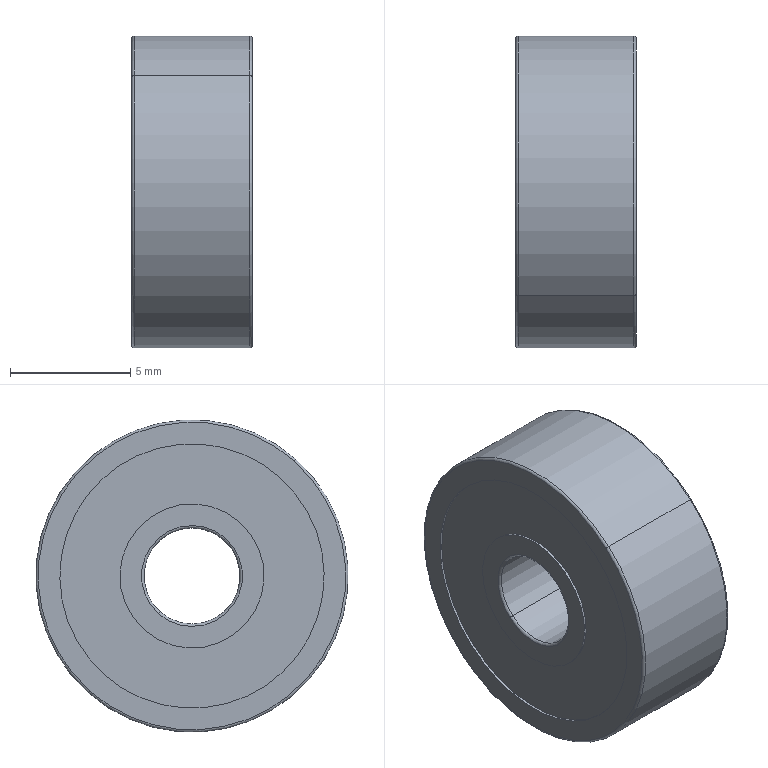Component | SolidWorks | DeepGrooveBallBearing624-2Z-1 | 1 solid | 26 faces | box 5 x 13 x 13 mm | volume 587 mm3 | cylinder 12 | torus 8 | plane 6 | commonest cylinder face diameters 11 x4 6 x4 13 x2 4 x2
build123d program:
from build123d import *

# Parameters (mm, degrees)
FILLET1_R = 0.1


with BuildPart() as part:
    # Sketch1 → Revolve1 (revolve)
    with BuildSketch(Plane.XY, mode=Mode.PRIVATE) as revolve1_sk:
        Polygon((-2.5, 6.5), (2.5, 6.5), (2.5, 5.5), (2.4, 5.5), (2.4, 3), (2.5, 3), (2.5, 2), (-2.5, 2), (-2.5, 3), (-2.4, 3), (-2.4, 5.5), (-2.5, 5.5), align=None)
    revolve(revolve1_sk.sketch.rotate(Axis((0, 0, 0), (1, 0, 0)), 90), axis=Axis((0, 0, 0), (1, 0, 0)))

    # Fillet1
    fillet1_edges = [part.edges().sort_by_distance(p)[0] for p in [
        (-2.5, 0, -2),
        (2.5, 0, -2),
        (2.5, 0, -6.5),
        (-2.5, 0, -6.5),
    ]]
    fillet(fillet1_edges, radius=FILLET1_R)


solid = part.part

# Placed as in the assembly
solid = solid.moved(Location((-0.3, -4.5, -27.446), (0, 0, 0)))
STEP:
#1=COLOUR_RGB('',0.7922,0.8196,0.9333);
#2=FILL_AREA_STYLE_COLOUR('',#1);
#3=FILL_AREA_STYLE('',(#2));
#4=SURFACE_STYLE_FILL_AREA(#3);
#5=SURFACE_SIDE_STYLE('',(#4));
#6=SURFACE_STYLE_USAGE(.BOTH.,#5);
#7=PRESENTATION_STYLE_ASSIGNMENT((#6));
#8=CARTESIAN_POINT('',(0.08661,-0.009757,-1.269));
#9=VERTEX_POINT('',#8);
#10=CARTESIAN_POINT('',(0.08661,-0.3446,-0.8922));
#11=VERTEX_POINT('',#10);
#12=CARTESIAN_POINT('',(0.08661,-0.1772,-1.081));
#13=DIRECTION('',(1.,-0.,-0.));
#14=DIRECTION('',(0.,-0.6644,0.7474));
#15=AXIS2_PLACEMENT_3D('',#12,#13,#14);
#16=CIRCLE('',#15,0.252);
#17=EDGE_CURVE('',#9,#11,#16,.T.);
#18=ORIENTED_EDGE('',*,*,#17,.F.);
#19=CARTESIAN_POINT('',(0.08268,-0.007141,-1.272));
#20=VERTEX_POINT('',#19);
#21=CARTESIAN_POINT('',(0.08268,-0.009757,-1.269));
#22=DIRECTION('',(0.,0.7474,0.6644));
#23=DIRECTION('',(0.,-0.6644,0.7474));
#24=AXIS2_PLACEMENT_3D('',#21,#22,#23);
#25=CIRCLE('',#24,0.003937);
#26=EDGE_CURVE('',#9,#20,#25,.T.);
#27=ORIENTED_EDGE('',*,*,#26,.T.);
#28=CARTESIAN_POINT('',(0.08268,-0.3472,-0.8893));
#29=VERTEX_POINT('',#28);
#30=CARTESIAN_POINT('',(0.08268,-0.1772,-1.081));
#31=DIRECTION('',(-1.,0.,0.));
#32=DIRECTION('',(0.,-0.6644,0.7474));
#33=AXIS2_PLACEMENT_3D('',#30,#31,#32);
#34=CIRCLE('',#33,0.2559);
#35=EDGE_CURVE('',#29,#20,#34,.T.);
#36=ORIENTED_EDGE('',*,*,#35,.F.);
#37=CARTESIAN_POINT('',(0.08268,-0.3446,-0.8922));
#38=DIRECTION('',(-0.,-0.7474,-0.6644));
#39=DIRECTION('',(0.,0.6644,-0.7474));
#40=AXIS2_PLACEMENT_3D('',#37,#38,#39);
#41=CIRCLE('',#40,0.003937);
#42=EDGE_CURVE('',#11,#29,#41,.T.);
#43=ORIENTED_EDGE('',*,*,#42,.F.);
#44=EDGE_LOOP('',(#18,#27,#36,#43));
#45=FACE_OUTER_BOUND('',#44,.T.);
#46=CARTESIAN_POINT('',(0.08268,-0.1772,-1.081));
#47=DIRECTION('',(-1.,0.,0.));
#48=DIRECTION('',(0.,-0.6644,0.7474));
#49=AXIS2_PLACEMENT_3D('',#46,#47,#48);
#50=TOROIDAL_SURFACE('',#49,0.252,0.003937);
#51=ADVANCED_FACE('',(#45),#50,.T.);
#52=CARTESIAN_POINT('',(-0.1102,-0.3446,-0.8922));
#53=VERTEX_POINT('',#52);
#54=CARTESIAN_POINT('',(-0.1102,-0.009757,-1.269));
#55=VERTEX_POINT('',#54);
#56=CARTESIAN_POINT('',(-0.1102,-0.1772,-1.081));
#57=DIRECTION('',(-1.,0.,0.));
#58=DIRECTION('',(0.,0.6644,-0.7474));
#59=AXIS2_PLACEMENT_3D('',#56,#57,#58);
#60=CIRCLE('',#59,0.252);
#61=EDGE_CURVE('',#53,#55,#60,.T.);
#62=ORIENTED_EDGE('',*,*,#61,.F.);
#63=CARTESIAN_POINT('',(-0.1063,-0.3472,-0.8893));
#64=VERTEX_POINT('',#63);
#65=CARTESIAN_POINT('',(-0.1063,-0.3446,-0.8922));
#66=DIRECTION('',(0.,0.7474,0.6644));
#67=DIRECTION('',(0.,-0.6644,0.7474));
#68=AXIS2_PLACEMENT_3D('',#65,#66,#67);
#69=CIRCLE('',#68,0.003937);
#70=EDGE_CURVE('',#53,#64,#69,.T.);
#71=ORIENTED_EDGE('',*,*,#70,.T.);
#72=CARTESIAN_POINT('',(-0.1063,-0.007141,-1.272));
#73=VERTEX_POINT('',#72);
#74=CARTESIAN_POINT('',(-0.1063,-0.1772,-1.081));
#75=DIRECTION('',(1.,-0.,-0.));
#76=DIRECTION('',(0.,0.6644,-0.7474));
#77=AXIS2_PLACEMENT_3D('',#74,#75,#76);
#78=CIRCLE('',#77,0.2559);
#79=EDGE_CURVE('',#73,#64,#78,.T.);
#80=ORIENTED_EDGE('',*,*,#79,.F.);
#81=CARTESIAN_POINT('',(-0.1063,-0.009757,-1.269));
#82=DIRECTION('',(-0.,-0.7474,-0.6644));
#83=DIRECTION('',(0.,0.6644,-0.7474));
#84=AXIS2_PLACEMENT_3D('',#81,#82,#83);
#85=CIRCLE('',#84,0.003937);
#86=EDGE_CURVE('',#55,#73,#85,.T.);
#87=ORIENTED_EDGE('',*,*,#86,.F.);
#88=EDGE_LOOP('',(#62,#71,#80,#87));
#89=FACE_OUTER_BOUND('',#88,.T.);
#90=CARTESIAN_POINT('',(-0.1063,-0.1772,-1.081));
#91=DIRECTION('',(1.,-0.,-0.));
#92=DIRECTION('',(-0.,0.6644,-0.7474));
#93=AXIS2_PLACEMENT_3D('',#90,#91,#92);
#94=TOROIDAL_SURFACE('',#93,0.252,0.003937);
#95=ADVANCED_FACE('',(#89),#94,.T.);
#96=CARTESIAN_POINT('',(0.08268,-0.1249,-1.139));
#97=VERTEX_POINT('',#96);
#98=CARTESIAN_POINT('',(0.08268,-0.2295,-1.022));
#99=VERTEX_POINT('',#98);
#100=CARTESIAN_POINT('',(0.08268,-0.1772,-1.081));
#101=DIRECTION('',(1.,-0.,-0.));
#102=DIRECTION('',(0.,-0.6644,0.7474));
#103=AXIS2_PLACEMENT_3D('',#100,#101,#102);
#104=CIRCLE('',#103,0.07874);
#105=EDGE_CURVE('',#97,#99,#104,.T.);
#106=ORIENTED_EDGE('',*,*,#105,.F.);
#107=CARTESIAN_POINT('',(0.08661,-0.1222,-1.142));
#108=VERTEX_POINT('',#107);
#109=CARTESIAN_POINT('',(0.08268,-0.1222,-1.142));
#110=DIRECTION('',(0.,0.7474,0.6644));
#111=DIRECTION('',(0.,-0.6644,0.7474));
#112=AXIS2_PLACEMENT_3D('',#109,#110,#111);
#113=CIRCLE('',#112,0.003937);
#114=EDGE_CURVE('',#97,#108,#113,.T.);
#115=ORIENTED_EDGE('',*,*,#114,.T.);
#116=CARTESIAN_POINT('',(0.08661,-0.2321,-1.019));
#117=VERTEX_POINT('',#116);
#118=CARTESIAN_POINT('',(0.08661,-0.1772,-1.081));
#119=DIRECTION('',(-1.,0.,0.));
#120=DIRECTION('',(0.,-0.6644,0.7474));
#121=AXIS2_PLACEMENT_3D('',#118,#119,#120);
#122=CIRCLE('',#121,0.08268);
#123=EDGE_CURVE('',#117,#108,#122,.T.);
#124=ORIENTED_EDGE('',*,*,#123,.F.);
#125=CARTESIAN_POINT('',(0.08268,-0.2321,-1.019));
#126=DIRECTION('',(-0.,-0.7474,-0.6644));
#127=DIRECTION('',(0.,0.6644,-0.7474));
#128=AXIS2_PLACEMENT_3D('',#125,#126,#127);
#129=CIRCLE('',#128,0.003937);
#130=EDGE_CURVE('',#99,#117,#129,.T.);
#131=ORIENTED_EDGE('',*,*,#130,.F.);
#132=EDGE_LOOP('',(#106,#115,#124,#131));
#133=FACE_OUTER_BOUND('',#132,.T.);
#134=CARTESIAN_POINT('',(0.08268,-0.1772,-1.081));
#135=DIRECTION('',(-1.,0.,0.));
#136=DIRECTION('',(0.,-0.6644,0.7474));
#137=AXIS2_PLACEMENT_3D('',#134,#135,#136);
#138=TOROIDAL_SURFACE('',#137,0.08268,0.003937);
#139=ADVANCED_FACE('',(#133),#138,.T.);
#140=CARTESIAN_POINT('',(-0.1063,-0.2295,-1.022));
#141=VERTEX_POINT('',#140);
#142=CARTESIAN_POINT('',(-0.1063,-0.1249,-1.139));
#143=VERTEX_POINT('',#142);
#144=CARTESIAN_POINT('',(-0.1063,-0.1772,-1.081));
#145=DIRECTION('',(-1.,0.,0.));
#146=DIRECTION('',(0.,0.6644,-0.7474));
#147=AXIS2_PLACEMENT_3D('',#144,#145,#146);
#148=CIRCLE('',#147,0.07874);
#149=EDGE_CURVE('',#141,#143,#148,.T.);
#150=ORIENTED_EDGE('',*,*,#149,.F.);
#151=CARTESIAN_POINT('',(-0.1102,-0.2321,-1.019));
#152=VERTEX_POINT('',#151);
#153=CARTESIAN_POINT('',(-0.1063,-0.2321,-1.019));
#154=DIRECTION('',(0.,0.7474,0.6644));
#155=DIRECTION('',(0.,-0.6644,0.7474));
#156=AXIS2_PLACEMENT_3D('',#153,#154,#155);
#157=CIRCLE('',#156,0.003937);
#158=EDGE_CURVE('',#141,#152,#157,.T.);
#159=ORIENTED_EDGE('',*,*,#158,.T.);
#160=CARTESIAN_POINT('',(-0.1102,-0.1222,-1.142));
#161=VERTEX_POINT('',#160);
#162=CARTESIAN_POINT('',(-0.1102,-0.1772,-1.081));
#163=DIRECTION('',(1.,-0.,-0.));
#164=DIRECTION('',(0.,0.6644,-0.7474));
#165=AXIS2_PLACEMENT_3D('',#162,#163,#164);
#166=CIRCLE('',#165,0.08268);
#167=EDGE_CURVE('',#161,#152,#166,.T.);
#168=ORIENTED_EDGE('',*,*,#167,.F.);
#169=CARTESIAN_POINT('',(-0.1063,-0.1222,-1.142));
#170=DIRECTION('',(-0.,-0.7474,-0.6644));
#171=DIRECTION('',(0.,0.6644,-0.7474));
#172=AXIS2_PLACEMENT_3D('',#169,#170,#171);
#173=CIRCLE('',#172,0.003937);
#174=EDGE_CURVE('',#143,#161,#173,.T.);
#175=ORIENTED_EDGE('',*,*,#174,.F.);
#176=EDGE_LOOP('',(#150,#159,#168,#175));
#177=FACE_OUTER_BOUND('',#176,.T.);
#178=CARTESIAN_POINT('',(-0.1063,-0.1772,-1.081));
#179=DIRECTION('',(1.,-0.,-0.));
#180=DIRECTION('',(-0.,0.6644,-0.7474));
#181=AXIS2_PLACEMENT_3D('',#178,#179,#180);
#182=TOROIDAL_SURFACE('',#181,0.08268,0.003937);
#183=ADVANCED_FACE('',(#177),#182,.T.);
#184=ORIENTED_EDGE('',*,*,#35,.T.);
#185=CARTESIAN_POINT('',(-0.01181,-0.007141,-1.272));
#186=DIRECTION('',(-1.,0.,0.));
#187=VECTOR('',#186,39.37);
#188=LINE('',#185,#187);
#189=EDGE_CURVE('',#20,#73,#188,.T.);
#190=ORIENTED_EDGE('',*,*,#189,.T.);
#191=ORIENTED_EDGE('',*,*,#79,.T.);
#192=CARTESIAN_POINT('',(-0.01181,-0.3472,-0.8893));
#193=DIRECTION('',(-1.,0.,0.));
#194=VECTOR('',#193,39.37);
#195=LINE('',#192,#194);
#196=EDGE_CURVE('',#29,#64,#195,.T.);
#197=ORIENTED_EDGE('',*,*,#196,.F.);
#198=EDGE_LOOP('',(#184,#190,#191,#197));
#199=FACE_OUTER_BOUND('',#198,.T.);
#200=CARTESIAN_POINT('',(-0.01181,-0.1772,-1.081));
#201=DIRECTION('',(-1.,0.,0.));
#202=DIRECTION('',(0.,-0.6644,0.7474));
#203=AXIS2_PLACEMENT_3D('',#200,#201,#202);
#204=CYLINDRICAL_SURFACE('',#203,0.2559);
#205=ADVANCED_FACE('',(#199),#204,.T.);
#206=CARTESIAN_POINT('',(-0.1063,-0.0333,-1.242));
#207=VERTEX_POINT('',#206);
#208=CARTESIAN_POINT('',(-0.1063,-0.321,-0.9187));
#209=VERTEX_POINT('',#208);
#210=CARTESIAN_POINT('',(-0.1063,-0.1772,-1.081));
#211=DIRECTION('',(-1.,0.,0.));
#212=DIRECTION('',(0.,-0.6644,0.7474));
#213=AXIS2_PLACEMENT_3D('',#210,#211,#212);
#214=CIRCLE('',#213,0.2165);
#215=EDGE_CURVE('',#207,#209,#214,.T.);
#216=ORIENTED_EDGE('',*,*,#215,.F.);
#217=CARTESIAN_POINT('',(-0.1102,-0.0333,-1.242));
#218=VERTEX_POINT('',#217);
#219=CARTESIAN_POINT('',(-0.01181,-0.0333,-1.242));
#220=DIRECTION('',(-1.,0.,0.));
#221=VECTOR('',#220,39.37);
#222=LINE('',#219,#221);
#223=EDGE_CURVE('',#207,#218,#222,.T.);
#224=ORIENTED_EDGE('',*,*,#223,.T.);
#225=CARTESIAN_POINT('',(-0.1102,-0.321,-0.9187));
#226=VERTEX_POINT('',#225);
#227=CARTESIAN_POINT('',(-0.1102,-0.1772,-1.081));
#228=DIRECTION('',(-1.,0.,0.));
#229=DIRECTION('',(0.,-0.6644,0.7474));
#230=AXIS2_PLACEMENT_3D('',#227,#228,#229);
#231=CIRCLE('',#230,0.2165);
#232=EDGE_CURVE('',#218,#226,#231,.T.);
#233=ORIENTED_EDGE('',*,*,#232,.T.);
#234=CARTESIAN_POINT('',(-0.01181,-0.321,-0.9187));
#235=DIRECTION('',(-1.,0.,0.));
#236=VECTOR('',#235,39.37);
#237=LINE('',#234,#236);
#238=EDGE_CURVE('',#209,#226,#237,.T.);
#239=ORIENTED_EDGE('',*,*,#238,.F.);
#240=EDGE_LOOP('',(#216,#224,#233,#239));
#241=FACE_OUTER_BOUND('',#240,.T.);
#242=CARTESIAN_POINT('',(-0.01181,-0.1772,-1.081));
#243=DIRECTION('',(-1.,0.,0.));
#244=DIRECTION('',(0.,-0.6644,0.7474));
#245=AXIS2_PLACEMENT_3D('',#242,#243,#244);
#246=CYLINDRICAL_SURFACE('',#245,0.2165);
#247=ADVANCED_FACE('',(#241),#246,.F.);
#248=CARTESIAN_POINT('',(-0.1063,-0.2556,-0.9923));
#249=VERTEX_POINT('',#248);
#250=CARTESIAN_POINT('',(-0.1063,-0.09869,-1.169));
#251=VERTEX_POINT('',#250);
#252=CARTESIAN_POINT('',(-0.1063,-0.1772,-1.081));
#253=DIRECTION('',(-1.,0.,0.));
#254=DIRECTION('',(0.,-0.6644,0.7474));
#255=AXIS2_PLACEMENT_3D('',#252,#253,#254);
#256=CIRCLE('',#255,0.1181);
#257=EDGE_CURVE('',#249,#251,#256,.T.);
#258=ORIENTED_EDGE('',*,*,#257,.T.);
#259=CARTESIAN_POINT('',(-0.1102,-0.09869,-1.169));
#260=VERTEX_POINT('',#259);
#261=CARTESIAN_POINT('',(-0.01181,-0.09869,-1.169));
#262=DIRECTION('',(-1.,0.,0.));
#263=VECTOR('',#262,39.37);
#264=LINE('',#261,#263);
#265=EDGE_CURVE('',#251,#260,#264,.T.);
#266=ORIENTED_EDGE('',*,*,#265,.T.);
#267=CARTESIAN_POINT('',(-0.1102,-0.2556,-0.9923));
#268=VERTEX_POINT('',#267);
#269=CARTESIAN_POINT('',(-0.1102,-0.1772,-1.081));
#270=DIRECTION('',(-1.,0.,0.));
#271=DIRECTION('',(0.,-0.6644,0.7474));
#272=AXIS2_PLACEMENT_3D('',#269,#270,#271);
#273=CIRCLE('',#272,0.1181);
#274=EDGE_CURVE('',#268,#260,#273,.T.);
#275=ORIENTED_EDGE('',*,*,#274,.F.);
#276=CARTESIAN_POINT('',(-0.01181,-0.2556,-0.9923));
#277=DIRECTION('',(-1.,0.,0.));
#278=VECTOR('',#277,39.37);
#279=LINE('',#276,#278);
#280=EDGE_CURVE('',#249,#268,#279,.T.);
#281=ORIENTED_EDGE('',*,*,#280,.F.);
#282=EDGE_LOOP('',(#258,#266,#275,#281));
#283=FACE_OUTER_BOUND('',#282,.T.);
#284=CARTESIAN_POINT('',(-0.01181,-0.1772,-1.081));
#285=DIRECTION('',(-1.,0.,0.));
#286=DIRECTION('',(0.,-0.6644,0.7474));
#287=AXIS2_PLACEMENT_3D('',#284,#285,#286);
#288=CYLINDRICAL_SURFACE('',#287,0.1181);
#289=ADVANCED_FACE('',(#283),#288,.T.);
#290=CARTESIAN_POINT('',(0.08268,-0.1772,-1.081));
#291=DIRECTION('',(1.,-0.,-0.));
#292=DIRECTION('',(0.,-0.6644,0.7474));
#293=AXIS2_PLACEMENT_3D('',#290,#291,#292);
#294=CIRCLE('',#293,0.07874);
#295=EDGE_CURVE('',#99,#97,#294,.T.);
#296=ORIENTED_EDGE('',*,*,#295,.T.);
#297=CARTESIAN_POINT('',(-0.01181,-0.1249,-1.139));
#298=DIRECTION('',(-1.,0.,0.));
#299=VECTOR('',#298,39.37);
#300=LINE('',#297,#299);
#301=EDGE_CURVE('',#97,#143,#300,.T.);
#302=ORIENTED_EDGE('',*,*,#301,.T.);
#303=CARTESIAN_POINT('',(-0.1063,-0.1772,-1.081));
#304=DIRECTION('',(-1.,0.,0.));
#305=DIRECTION('',(0.,0.6644,-0.7474));
#306=AXIS2_PLACEMENT_3D('',#303,#304,#305);
#307=CIRCLE('',#306,0.07874);
#308=EDGE_CURVE('',#143,#141,#307,.T.);
#309=ORIENTED_EDGE('',*,*,#308,.T.);
#310=CARTESIAN_POINT('',(-0.01181,-0.2295,-1.022));
#311=DIRECTION('',(-1.,0.,0.));
#312=VECTOR('',#311,39.37);
#313=LINE('',#310,#312);
#314=EDGE_CURVE('',#99,#141,#313,.T.);
#315=ORIENTED_EDGE('',*,*,#314,.F.);
#316=EDGE_LOOP('',(#296,#302,#309,#315));
#317=FACE_OUTER_BOUND('',#316,.T.);
#318=CARTESIAN_POINT('',(-0.01181,-0.1772,-1.081));
#319=DIRECTION('',(-1.,0.,0.));
#320=DIRECTION('',(0.,-0.6644,0.7474));
#321=AXIS2_PLACEMENT_3D('',#318,#319,#320);
#322=CYLINDRICAL_SURFACE('',#321,0.07874);
#323=ADVANCED_FACE('',(#317),#322,.F.);
#324=CARTESIAN_POINT('',(0.08661,-0.2556,-0.9923));
#325=VERTEX_POINT('',#324);
#326=CARTESIAN_POINT('',(0.08661,-0.09869,-1.169));
#327=VERTEX_POINT('',#326);
#328=CARTESIAN_POINT('',(0.08661,-0.1772,-1.081));
#329=DIRECTION('',(-1.,0.,0.));
#330=DIRECTION('',(0.,-0.6644,0.7474));
#331=AXIS2_PLACEMENT_3D('',#328,#329,#330);
#332=CIRCLE('',#331,0.1181);
#333=EDGE_CURVE('',#325,#327,#332,.T.);
#334=ORIENTED_EDGE('',*,*,#333,.T.);
#335=CARTESIAN_POINT('',(0.08268,-0.09869,-1.169));
#336=VERTEX_POINT('',#335);
#337=CARTESIAN_POINT('',(-0.01181,-0.09869,-1.169));
#338=DIRECTION('',(-1.,0.,0.));
#339=VECTOR('',#338,39.37);
#340=LINE('',#337,#339);
#341=EDGE_CURVE('',#327,#336,#340,.T.);
#342=ORIENTED_EDGE('',*,*,#341,.T.);
#343=CARTESIAN_POINT('',(0.08268,-0.2556,-0.9923));
#344=VERTEX_POINT('',#343);
#345=CARTESIAN_POINT('',(0.08268,-0.1772,-1.081));
#346=DIRECTION('',(-1.,0.,0.));
#347=DIRECTION('',(0.,-0.6644,0.7474));
#348=AXIS2_PLACEMENT_3D('',#345,#346,#347);
#349=CIRCLE('',#348,0.1181);
#350=EDGE_CURVE('',#344,#336,#349,.T.);
#351=ORIENTED_EDGE('',*,*,#350,.F.);
#352=CARTESIAN_POINT('',(-0.01181,-0.2556,-0.9923));
#353=DIRECTION('',(-1.,0.,0.));
#354=VECTOR('',#353,39.37);
#355=LINE('',#352,#354);
#356=EDGE_CURVE('',#325,#344,#355,.T.);
#357=ORIENTED_EDGE('',*,*,#356,.F.);
#358=EDGE_LOOP('',(#334,#342,#351,#357));
#359=FACE_OUTER_BOUND('',#358,.T.);
#360=CARTESIAN_POINT('',(-0.01181,-0.1772,-1.081));
#361=DIRECTION('',(-1.,0.,0.));
#362=DIRECTION('',(0.,-0.6644,0.7474));
#363=AXIS2_PLACEMENT_3D('',#360,#361,#362);
#364=CYLINDRICAL_SURFACE('',#363,0.1181);
#365=ADVANCED_FACE('',(#359),#364,.T.);
#366=CARTESIAN_POINT('',(0.08661,-0.0333,-1.242));
#367=VERTEX_POINT('',#366);
#368=CARTESIAN_POINT('',(0.08661,-0.321,-0.9187));
#369=VERTEX_POINT('',#368);
#370=CARTESIAN_POINT('',(0.08661,-0.1772,-1.081));
#371=DIRECTION('',(-1.,0.,0.));
#372=DIRECTION('',(0.,-0.6644,0.7474));
#373=AXIS2_PLACEMENT_3D('',#370,#371,#372);
#374=CIRCLE('',#373,0.2165);
#375=EDGE_CURVE('',#367,#369,#374,.T.);
#376=ORIENTED_EDGE('',*,*,#375,.F.);
#377=CARTESIAN_POINT('',(0.08268,-0.0333,-1.242));
#378=VERTEX_POINT('',#377);
#379=CARTESIAN_POINT('',(-0.01181,-0.0333,-1.242));
#380=DIRECTION('',(-1.,0.,0.));
#381=VECTOR('',#380,39.37);
#382=LINE('',#379,#381);
#383=EDGE_CURVE('',#367,#378,#382,.T.);
#384=ORIENTED_EDGE('',*,*,#383,.T.);
#385=CARTESIAN_POINT('',(0.08268,-0.321,-0.9187));
#386=VERTEX_POINT('',#385);
#387=CARTESIAN_POINT('',(0.08268,-0.1772,-1.081));
#388=DIRECTION('',(-1.,0.,0.));
#389=DIRECTION('',(0.,-0.6644,0.7474));
#390=AXIS2_PLACEMENT_3D('',#387,#388,#389);
#391=CIRCLE('',#390,0.2165);
#392=EDGE_CURVE('',#378,#386,#391,.T.);
#393=ORIENTED_EDGE('',*,*,#392,.T.);
#394=CARTESIAN_POINT('',(-0.01181,-0.321,-0.9187));
#395=DIRECTION('',(-1.,0.,0.));
#396=VECTOR('',#395,39.37);
#397=LINE('',#394,#396);
#398=EDGE_CURVE('',#369,#386,#397,.T.);
#399=ORIENTED_EDGE('',*,*,#398,.F.);
#400=EDGE_LOOP('',(#376,#384,#393,#399));
#401=FACE_OUTER_BOUND('',#400,.T.);
#402=CARTESIAN_POINT('',(-0.01181,-0.1772,-1.081));
#403=DIRECTION('',(-1.,0.,0.));
#404=DIRECTION('',(0.,-0.6644,0.7474));
#405=AXIS2_PLACEMENT_3D('',#402,#403,#404);
#406=CYLINDRICAL_SURFACE('',#405,0.2165);
#407=ADVANCED_FACE('',(#401),#406,.F.);
#408=CARTESIAN_POINT('',(0.08661,-0.1772,-1.081));
#409=DIRECTION('',(1.,-0.,-0.));
#410=DIRECTION('',(0.,-0.6644,0.7474));
#411=AXIS2_PLACEMENT_3D('',#408,#409,#410);
#412=CIRCLE('',#411,0.252);
#413=EDGE_CURVE('',#11,#9,#412,.T.);
#414=ORIENTED_EDGE('',*,*,#413,.T.);
#415=ORIENTED_EDGE('',*,*,#17,.T.);
#416=EDGE_LOOP('',(#414,#415));
#417=FACE_OUTER_BOUND('',#416,.T.);
#418=CARTESIAN_POINT('',(0.08661,-0.1772,-1.081));
#419=DIRECTION('',(-1.,0.,0.));
#420=DIRECTION('',(0.,-0.6644,0.7474));
#421=AXIS2_PLACEMENT_3D('',#418,#419,#420);
#422=CIRCLE('',#421,0.2165);
#423=EDGE_CURVE('',#369,#367,#422,.T.);
#424=ORIENTED_EDGE('',*,*,#423,.T.);
#425=ORIENTED_EDGE('',*,*,#375,.T.);
#426=EDGE_LOOP('',(#424,#425));
#427=FACE_BOUND('',#426,.T.);
#428=CARTESIAN_POINT('',(0.08661,0.01409,-0.9105));
#429=DIRECTION('',(-1.,0.,0.));
#430=DIRECTION('',(0.,-0.6644,0.7474));
#431=AXIS2_PLACEMENT_3D('',#428,#429,#430);
#432=PLANE('',#431);
#433=ADVANCED_FACE('',(#417,#427),#432,.F.);
#434=ORIENTED_EDGE('',*,*,#383,.F.);
#435=ORIENTED_EDGE('',*,*,#423,.F.);
#436=ORIENTED_EDGE('',*,*,#398,.T.);
#437=CARTESIAN_POINT('',(0.08268,-0.1772,-1.081));
#438=DIRECTION('',(-1.,0.,0.));
#439=DIRECTION('',(0.,-0.6644,0.7474));
#440=AXIS2_PLACEMENT_3D('',#437,#438,#439);
#441=CIRCLE('',#440,0.2165);
#442=EDGE_CURVE('',#386,#378,#441,.T.);
#443=ORIENTED_EDGE('',*,*,#442,.T.);
#444=EDGE_LOOP('',(#434,#435,#436,#443));
#445=FACE_OUTER_BOUND('',#444,.T.);
#446=CARTESIAN_POINT('',(-0.01181,-0.1772,-1.081));
#447=DIRECTION('',(-1.,0.,0.));
#448=DIRECTION('',(0.,-0.6644,0.7474));
#449=AXIS2_PLACEMENT_3D('',#446,#447,#448);
#450=CYLINDRICAL_SURFACE('',#449,0.2165);
#451=ADVANCED_FACE('',(#445),#450,.F.);
#452=ORIENTED_EDGE('',*,*,#442,.F.);
#453=ORIENTED_EDGE('',*,*,#392,.F.);
#454=EDGE_LOOP('',(#452,#453));
#455=FACE_OUTER_BOUND('',#454,.T.);
#456=ORIENTED_EDGE('',*,*,#350,.T.);
#457=CARTESIAN_POINT('',(0.08268,-0.1772,-1.081));
#458=DIRECTION('',(-1.,0.,0.));
#459=DIRECTION('',(0.,-0.6644,0.7474));
#460=AXIS2_PLACEMENT_3D('',#457,#458,#459);
#461=CIRCLE('',#460,0.1181);
#462=EDGE_CURVE('',#336,#344,#461,.T.);
#463=ORIENTED_EDGE('',*,*,#462,.T.);
#464=EDGE_LOOP('',(#456,#463));
#465=FACE_BOUND('',#464,.T.);
#466=CARTESIAN_POINT('',(0.08268,-0.01533,-0.9367));
#467=DIRECTION('',(-1.,0.,0.));
#468=DIRECTION('',(0.,-0.6644,0.7474));
#469=AXIS2_PLACEMENT_3D('',#466,#467,#468);
#470=PLANE('',#469);
#471=ADVANCED_FACE('',(#455,#465),#470,.F.);
#472=ORIENTED_EDGE('',*,*,#341,.F.);
#473=CARTESIAN_POINT('',(0.08661,-0.1772,-1.081));
#474=DIRECTION('',(-1.,0.,0.));
#475=DIRECTION('',(0.,-0.6644,0.7474));
#476=AXIS2_PLACEMENT_3D('',#473,#474,#475);
#477=CIRCLE('',#476,0.1181);
#478=EDGE_CURVE('',#327,#325,#477,.T.);
#479=ORIENTED_EDGE('',*,*,#478,.T.);
#480=ORIENTED_EDGE('',*,*,#356,.T.);
#481=ORIENTED_EDGE('',*,*,#462,.F.);
#482=EDGE_LOOP('',(#472,#479,#480,#481));
#483=FACE_OUTER_BOUND('',#482,.T.);
#484=CARTESIAN_POINT('',(-0.01181,-0.1772,-1.081));
#485=DIRECTION('',(-1.,0.,0.));
#486=DIRECTION('',(0.,-0.6644,0.7474));
#487=AXIS2_PLACEMENT_3D('',#484,#485,#486);
#488=CYLINDRICAL_SURFACE('',#487,0.1181);
#489=ADVANCED_FACE('',(#483),#488,.T.);
#490=ORIENTED_EDGE('',*,*,#123,.T.);
#491=CARTESIAN_POINT('',(0.08661,-0.1772,-1.081));
#492=DIRECTION('',(-1.,0.,0.));
#493=DIRECTION('',(0.,-0.6644,0.7474));
#494=AXIS2_PLACEMENT_3D('',#491,#492,#493);
#495=CIRCLE('',#494,0.08268);
#496=EDGE_CURVE('',#108,#117,#495,.T.);
#497=ORIENTED_EDGE('',*,*,#496,.T.);
#498=EDGE_LOOP('',(#490,#497));
#499=FACE_BOUND('',#498,.T.);
#500=ORIENTED_EDGE('',*,*,#333,.F.);
#501=ORIENTED_EDGE('',*,*,#478,.F.);
#502=EDGE_LOOP('',(#500,#501));
#503=FACE_OUTER_BOUND('',#502,.T.);
#504=CARTESIAN_POINT('',(0.08661,-0.08889,-1.002));
#505=DIRECTION('',(-1.,0.,0.));
#506=DIRECTION('',(0.,-0.6644,0.7474));
#507=AXIS2_PLACEMENT_3D('',#504,#505,#506);
#508=PLANE('',#507);
#509=ADVANCED_FACE('',(#499,#503),#508,.F.);
#510=ORIENTED_EDGE('',*,*,#301,.F.);
#511=ORIENTED_EDGE('',*,*,#105,.T.);
#512=ORIENTED_EDGE('',*,*,#314,.T.);
#513=ORIENTED_EDGE('',*,*,#149,.T.);
#514=EDGE_LOOP('',(#510,#511,#512,#513));
#515=FACE_OUTER_BOUND('',#514,.T.);
#516=CARTESIAN_POINT('',(-0.01181,-0.1772,-1.081));
#517=DIRECTION('',(-1.,0.,0.));
#518=DIRECTION('',(0.,-0.6644,0.7474));
#519=AXIS2_PLACEMENT_3D('',#516,#517,#518);
#520=CYLINDRICAL_SURFACE('',#519,0.07874);
#521=ADVANCED_FACE('',(#515),#520,.F.);
#522=ORIENTED_EDGE('',*,*,#167,.T.);
#523=CARTESIAN_POINT('',(-0.1102,-0.1772,-1.081));
#524=DIRECTION('',(1.,-0.,-0.));
#525=DIRECTION('',(0.,0.6644,-0.7474));
#526=AXIS2_PLACEMENT_3D('',#523,#524,#525);
#527=CIRCLE('',#526,0.08268);
#528=EDGE_CURVE('',#152,#161,#527,.T.);
#529=ORIENTED_EDGE('',*,*,#528,.T.);
#530=EDGE_LOOP('',(#522,#529));
#531=FACE_BOUND('',#530,.T.);
#532=ORIENTED_EDGE('',*,*,#274,.T.);
#533=CARTESIAN_POINT('',(-0.1102,-0.1772,-1.081));
#534=DIRECTION('',(-1.,0.,0.));
#535=DIRECTION('',(0.,-0.6644,0.7474));
#536=AXIS2_PLACEMENT_3D('',#533,#534,#535);
#537=CIRCLE('',#536,0.1181);
#538=EDGE_CURVE('',#260,#268,#537,.T.);
#539=ORIENTED_EDGE('',*,*,#538,.T.);
#540=EDGE_LOOP('',(#532,#539));
#541=FACE_OUTER_BOUND('',#540,.T.);
#542=CARTESIAN_POINT('',(-0.1102,-0.08889,-1.002));
#543=DIRECTION('',(1.,-0.,-0.));
#544=DIRECTION('',(-0.,0.6644,-0.7474));
#545=AXIS2_PLACEMENT_3D('',#542,#543,#544);
#546=PLANE('',#545);
#547=ADVANCED_FACE('',(#531,#541),#546,.F.);
#548=ORIENTED_EDGE('',*,*,#265,.F.);
#549=CARTESIAN_POINT('',(-0.1063,-0.1772,-1.081));
#550=DIRECTION('',(-1.,0.,0.));
#551=DIRECTION('',(0.,-0.6644,0.7474));
#552=AXIS2_PLACEMENT_3D('',#549,#550,#551);
#553=CIRCLE('',#552,0.1181);
#554=EDGE_CURVE('',#251,#249,#553,.T.);
#555=ORIENTED_EDGE('',*,*,#554,.T.);
#556=ORIENTED_EDGE('',*,*,#280,.T.);
#557=ORIENTED_EDGE('',*,*,#538,.F.);
#558=EDGE_LOOP('',(#548,#555,#556,#557));
#559=FACE_OUTER_BOUND('',#558,.T.);
#560=CARTESIAN_POINT('',(-0.01181,-0.1772,-1.081));
#561=DIRECTION('',(-1.,0.,0.));
#562=DIRECTION('',(0.,-0.6644,0.7474));
#563=AXIS2_PLACEMENT_3D('',#560,#561,#562);
#564=CYLINDRICAL_SURFACE('',#563,0.1181);
#565=ADVANCED_FACE('',(#559),#564,.T.);
#566=ORIENTED_EDGE('',*,*,#257,.F.);
#567=ORIENTED_EDGE('',*,*,#554,.F.);
#568=EDGE_LOOP('',(#566,#567));
#569=FACE_BOUND('',#568,.T.);
#570=CARTESIAN_POINT('',(-0.1063,-0.1772,-1.081));
#571=DIRECTION('',(-1.,0.,0.));
#572=DIRECTION('',(0.,-0.6644,0.7474));
#573=AXIS2_PLACEMENT_3D('',#570,#571,#572);
#574=CIRCLE('',#573,0.2165);
#575=EDGE_CURVE('',#209,#207,#574,.T.);
#576=ORIENTED_EDGE('',*,*,#575,.T.);
#577=ORIENTED_EDGE('',*,*,#215,.T.);
#578=EDGE_LOOP('',(#576,#577));
#579=FACE_OUTER_BOUND('',#578,.T.);
#580=CARTESIAN_POINT('',(-0.1063,-0.01533,-0.9367));
#581=DIRECTION('',(1.,-0.,-0.));
#582=DIRECTION('',(-0.,0.6644,-0.7474));
#583=AXIS2_PLACEMENT_3D('',#580,#581,#582);
#584=PLANE('',#583);
#585=ADVANCED_FACE('',(#569,#579),#584,.F.);
#586=ORIENTED_EDGE('',*,*,#223,.F.);
#587=ORIENTED_EDGE('',*,*,#575,.F.);
#588=ORIENTED_EDGE('',*,*,#238,.T.);
#589=CARTESIAN_POINT('',(-0.1102,-0.1772,-1.081));
#590=DIRECTION('',(-1.,0.,0.));
#591=DIRECTION('',(0.,-0.6644,0.7474));
#592=AXIS2_PLACEMENT_3D('',#589,#590,#591);
#593=CIRCLE('',#592,0.2165);
#594=EDGE_CURVE('',#226,#218,#593,.T.);
#595=ORIENTED_EDGE('',*,*,#594,.T.);
#596=EDGE_LOOP('',(#586,#587,#588,#595));
#597=FACE_OUTER_BOUND('',#596,.T.);
#598=CARTESIAN_POINT('',(-0.01181,-0.1772,-1.081));
#599=DIRECTION('',(-1.,0.,0.));
#600=DIRECTION('',(0.,-0.6644,0.7474));
#601=AXIS2_PLACEMENT_3D('',#598,#599,#600);
#602=CYLINDRICAL_SURFACE('',#601,0.2165);
#603=ADVANCED_FACE('',(#597),#602,.F.);
#604=CARTESIAN_POINT('',(-0.1102,-0.1772,-1.081));
#605=DIRECTION('',(-1.,0.,0.));
#606=DIRECTION('',(0.,0.6644,-0.7474));
#607=AXIS2_PLACEMENT_3D('',#604,#605,#606);
#608=CIRCLE('',#607,0.252);
#609=EDGE_CURVE('',#55,#53,#608,.T.);
#610=ORIENTED_EDGE('',*,*,#609,.T.);
#611=ORIENTED_EDGE('',*,*,#61,.T.);
#612=EDGE_LOOP('',(#610,#611));
#613=FACE_OUTER_BOUND('',#612,.T.);
#614=ORIENTED_EDGE('',*,*,#594,.F.);
#615=ORIENTED_EDGE('',*,*,#232,.F.);
#616=EDGE_LOOP('',(#614,#615));
#617=FACE_BOUND('',#616,.T.);
#618=CARTESIAN_POINT('',(-0.1102,0.01409,-0.9105));
#619=DIRECTION('',(1.,-0.,-0.));
#620=DIRECTION('',(-0.,0.6644,-0.7474));
#621=AXIS2_PLACEMENT_3D('',#618,#619,#620);
#622=PLANE('',#621);
#623=ADVANCED_FACE('',(#613,#617),#622,.F.);
#624=ORIENTED_EDGE('',*,*,#189,.F.);
#625=CARTESIAN_POINT('',(0.08268,-0.1772,-1.081));
#626=DIRECTION('',(-1.,0.,0.));
#627=DIRECTION('',(0.,-0.6644,0.7474));
#628=AXIS2_PLACEMENT_3D('',#625,#626,#627);
#629=CIRCLE('',#628,0.2559);
#630=EDGE_CURVE('',#20,#29,#629,.T.);
#631=ORIENTED_EDGE('',*,*,#630,.T.);
#632=ORIENTED_EDGE('',*,*,#196,.T.);
#633=CARTESIAN_POINT('',(-0.1063,-0.1772,-1.081));
#634=DIRECTION('',(1.,-0.,-0.));
#635=DIRECTION('',(0.,0.6644,-0.7474));
#636=AXIS2_PLACEMENT_3D('',#633,#634,#635);
#637=CIRCLE('',#636,0.2559);
#638=EDGE_CURVE('',#64,#73,#637,.T.);
#639=ORIENTED_EDGE('',*,*,#638,.T.);
#640=EDGE_LOOP('',(#624,#631,#632,#639));
#641=FACE_OUTER_BOUND('',#640,.T.);
#642=CARTESIAN_POINT('',(-0.01181,-0.1772,-1.081));
#643=DIRECTION('',(-1.,0.,0.));
#644=DIRECTION('',(0.,-0.6644,0.7474));
#645=AXIS2_PLACEMENT_3D('',#642,#643,#644);
#646=CYLINDRICAL_SURFACE('',#645,0.2559);
#647=ADVANCED_FACE('',(#641),#646,.T.);
#648=ORIENTED_EDGE('',*,*,#158,.F.);
#649=ORIENTED_EDGE('',*,*,#308,.F.);
#650=ORIENTED_EDGE('',*,*,#174,.T.);
#651=ORIENTED_EDGE('',*,*,#528,.F.);
#652=EDGE_LOOP('',(#648,#649,#650,#651));
#653=FACE_OUTER_BOUND('',#652,.T.);
#654=CARTESIAN_POINT('',(-0.1063,-0.1772,-1.081));
#655=DIRECTION('',(1.,-0.,-0.));
#656=DIRECTION('',(-0.,0.6644,-0.7474));
#657=AXIS2_PLACEMENT_3D('',#654,#655,#656);
#658=TOROIDAL_SURFACE('',#657,0.08268,0.003937);
#659=ADVANCED_FACE('',(#653),#658,.T.);
#660=ORIENTED_EDGE('',*,*,#114,.F.);
#661=ORIENTED_EDGE('',*,*,#295,.F.);
#662=ORIENTED_EDGE('',*,*,#130,.T.);
#663=ORIENTED_EDGE('',*,*,#496,.F.);
#664=EDGE_LOOP('',(#660,#661,#662,#663));
#665=FACE_OUTER_BOUND('',#664,.T.);
#666=CARTESIAN_POINT('',(0.08268,-0.1772,-1.081));
#667=DIRECTION('',(-1.,0.,0.));
#668=DIRECTION('',(0.,-0.6644,0.7474));
#669=AXIS2_PLACEMENT_3D('',#666,#667,#668);
#670=TOROIDAL_SURFACE('',#669,0.08268,0.003937);
#671=ADVANCED_FACE('',(#665),#670,.T.);
#672=ORIENTED_EDGE('',*,*,#70,.F.);
#673=ORIENTED_EDGE('',*,*,#609,.F.);
#674=ORIENTED_EDGE('',*,*,#86,.T.);
#675=ORIENTED_EDGE('',*,*,#638,.F.);
#676=EDGE_LOOP('',(#672,#673,#674,#675));
#677=FACE_OUTER_BOUND('',#676,.T.);
#678=CARTESIAN_POINT('',(-0.1063,-0.1772,-1.081));
#679=DIRECTION('',(1.,-0.,-0.));
#680=DIRECTION('',(-0.,0.6644,-0.7474));
#681=AXIS2_PLACEMENT_3D('',#678,#679,#680);
#682=TOROIDAL_SURFACE('',#681,0.252,0.003937);
#683=ADVANCED_FACE('',(#677),#682,.T.);
#684=ORIENTED_EDGE('',*,*,#26,.F.);
#685=ORIENTED_EDGE('',*,*,#413,.F.);
#686=ORIENTED_EDGE('',*,*,#42,.T.);
#687=ORIENTED_EDGE('',*,*,#630,.F.);
#688=EDGE_LOOP('',(#684,#685,#686,#687));
#689=FACE_OUTER_BOUND('',#688,.T.);
#690=CARTESIAN_POINT('',(0.08268,-0.1772,-1.081));
#691=DIRECTION('',(-1.,0.,0.));
#692=DIRECTION('',(0.,-0.6644,0.7474));
#693=AXIS2_PLACEMENT_3D('',#690,#691,#692);
#694=TOROIDAL_SURFACE('',#693,0.252,0.003937);
#695=ADVANCED_FACE('',(#689),#694,.T.);
#696=CLOSED_SHELL('',(#51,#95,#139,#183,#205,#247,#289,#323,#365,#407,#433,#451,#471,#489,#509,#521,#547,#565,#585,#603,#623,#647,#659,#671,#683,#695));
#697=MANIFOLD_SOLID_BREP('',#696);
#698=STYLED_ITEM('',(#7),#697);
#699=PRESENTATION_LAYER_ASSIGNMENT('','',(#698));
#700=CARTESIAN_POINT('',(0.,0.,0.));
#701=DIRECTION('',(0.,0.,1.));
#702=DIRECTION('',(1.,0.,0.));
#703=AXIS2_PLACEMENT_3D('',#700,#701,#702);
#704=(LENGTH_UNIT()NAMED_UNIT(*)SI_UNIT($,.METRE.));
#705=LENGTH_MEASURE_WITH_UNIT(LENGTH_MEASURE(0.0254),#704);
#706=DIMENSIONAL_EXPONENTS(1.,0.,0.,0.,0.,0.,0.);
#707=(CONVERSION_BASED_UNIT('',#705)LENGTH_UNIT()NAMED_UNIT(#706));
#708=UNCERTAINTY_MEASURE_WITH_UNIT(LENGTH_MEASURE(0.00001),#707,'','');
#709=(NAMED_UNIT(*)PLANE_ANGLE_UNIT()SI_UNIT($,.RADIAN.));
#710=(NAMED_UNIT(*)SI_UNIT($,.STERADIAN.)SOLID_ANGLE_UNIT());
#711=(GEOMETRIC_REPRESENTATION_CONTEXT(3)GLOBAL_UNCERTAINTY_ASSIGNED_CONTEXT((#708))GLOBAL_UNIT_ASSIGNED_CONTEXT((#707,#709,#710))REPRESENTATION_CONTEXT('',''));
#712=ADVANCED_BREP_SHAPE_REPRESENTATION('',(#697,#703),#711);
#713=(LENGTH_UNIT()NAMED_UNIT(*)SI_UNIT($,.METRE.));
#714=LENGTH_MEASURE_WITH_UNIT(LENGTH_MEASURE(0.0254),#713);
#715=DIMENSIONAL_EXPONENTS(1.,0.,0.,0.,0.,0.,0.);
#716=(CONVERSION_BASED_UNIT('',#714)LENGTH_UNIT()NAMED_UNIT(#715));
#717=UNCERTAINTY_MEASURE_WITH_UNIT(LENGTH_MEASURE(0.00001),#716,'','');
#718=(NAMED_UNIT(*)PLANE_ANGLE_UNIT()SI_UNIT($,.RADIAN.));
#719=(NAMED_UNIT(*)SI_UNIT($,.STERADIAN.)SOLID_ANGLE_UNIT());
#720=(GEOMETRIC_REPRESENTATION_CONTEXT(3)GLOBAL_UNCERTAINTY_ASSIGNED_CONTEXT((#717))GLOBAL_UNIT_ASSIGNED_CONTEXT((#716,#718,#719))REPRESENTATION_CONTEXT('',''));
#721=MECHANICAL_DESIGN_GEOMETRIC_PRESENTATION_REPRESENTATION('',(#698),#720);